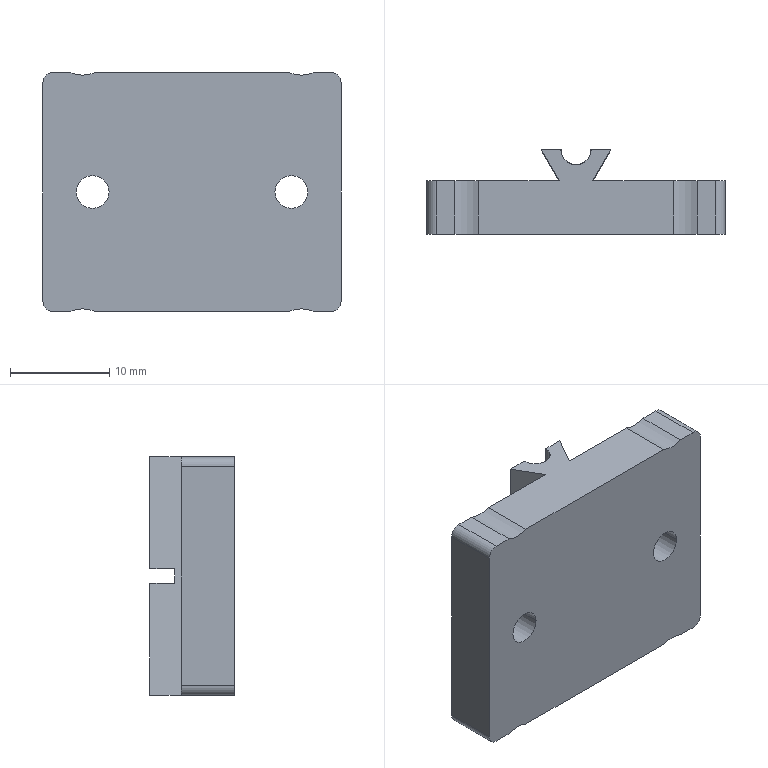Component | SolidWorks | Slider-3 | 1 solid | 39 faces | box 30 x 8.5 x 24 mm | volume 4033 mm3 | plane 20 | cylinder 14 | cone 5 | commonest cylinder face diameters 3.3 x4 2 x4 6 x4 3 x2
build123d program:
from build123d import *

# Parameters (mm, degrees)
SKETCH1_2_W                 = 24
SKETCH1_2_H                 = 30
BOSS_EXTRUDE1_DEPTH         = 10
M3_TAPPED_HOLE1_D           = 2.5
M3_TAPPED_HOLE1_CSINK_D     = 3.05
M3_TAPPED_HOLE1_CSINK_ANGLE = 100
CUT_EXTRUDE1_2_DEPTH        = 31.017
SKETCH6_W                   = 1.5
SKETCH6_H                   = 7
CUT_EXTRUDE4_DEPTH          = 4
FILLET1_R                   = 1
M4_TAPPED_HOLE3_D           = 3.3
M4_TAPPED_HOLE3_CSINK_D     = 4.05
M4_TAPPED_HOLE3_CSINK_ANGLE = 100
SKETCH1_R                   = 1.5
CUT_EXTRUDE1_DEPTH          = 24
SKETCH2_R                   = 3
CUT_EXTRUDE2_DEPTH          = 6


with BuildPart() as part:
    # Sketch1_2 → Boss-Extrude1 (new body)
    with BuildSketch(Plane(origin=(0, 0, 0), x_dir=(1, 0, 0), z_dir=(0, 1, 0))):
        Rectangle(SKETCH1_2_W, SKETCH1_2_H)
    extrude(amount=BOSS_EXTRUDE1_DEPTH)

    # M3 Tapped Hole1 (through all)
    with Locations(Plane(origin=(12, 8.5, 0), x_dir=(0, 0, 1), z_dir=(1, 0, 0))):
        with Locations((0, 0)):
            CounterSinkHole(M3_TAPPED_HOLE1_D / 2, M3_TAPPED_HOLE1_CSINK_D / 2, counter_sink_angle=M3_TAPPED_HOLE1_CSINK_ANGLE)

    # Sketch2_2 → Cut-Extrude1_2 (cut, through all)
    with BuildSketch(Plane(origin=(12, 0, 0), x_dir=(0, 0, -1), z_dir=(1, 0, 0))):
        Polygon((-15, 5.343), (-15, 10), (15, 10), (15, 5.343), (1.677, 5.343), (3.5, 8.5), (-3.5, 8.5), (-1.677, 5.343), align=None)
    extrude(amount=-CUT_EXTRUDE1_2_DEPTH, mode=Mode.SUBTRACT)

    # Sketch6 → Cut-Extrude4 (cut)
    with BuildSketch(Plane(origin=(0, 10, 0), x_dir=(1, 0, 0), z_dir=(0, 1, 0))):
        Rectangle(SKETCH6_W, SKETCH6_H)
    extrude(amount=-CUT_EXTRUDE4_DEPTH, mode=Mode.SUBTRACT)

    # Fillet1
    fillet1_edges = [part.edges().sort_by_distance(p)[0] for p in [
        (12, 2.671, 15),
        (-12, 2.671, 15),
        (-12, 2.671, -15),
        (12, 2.671, -15),
    ]]
    fillet(fillet1_edges, radius=FILLET1_R)

    # M4 Tapped Hole3 (through all)
    with Locations(Plane(origin=(0, 5.343, -10), x_dir=(0, 0, 1), z_dir=(0, 1, 0))):
        with Locations((0, 0), (20, 0)):
            CounterSinkHole(M4_TAPPED_HOLE3_D / 2, M4_TAPPED_HOLE3_CSINK_D / 2, counter_sink_angle=M4_TAPPED_HOLE3_CSINK_ANGLE)

    # Sketch1 → Cut-Extrude1 (cut)
    with BuildSketch(Plane(origin=(12, 0, 0), x_dir=(0, 0, -1), z_dir=(1, 0, 0))):
        with Locations((0, 8.5)):
            Circle(SKETCH1_R)
    extrude(amount=-CUT_EXTRUDE1_DEPTH, mode=Mode.SUBTRACT)

    # Sketch2 → Cut-Extrude2 (cut)
    with BuildSketch(Plane.XZ):
        with Locations((-14.755, 11)):
            Circle(SKETCH2_R)
        with Locations((-14.755, -11)):
            Circle(SKETCH2_R)
        with Locations((14.755, 11)):
            Circle(SKETCH2_R)
        with Locations((14.755, -11)):
            Circle(SKETCH2_R)
    extrude(amount=-CUT_EXTRUDE2_DEPTH, mode=Mode.SUBTRACT)


solid = part.part

# Placed as in the assembly
solid = solid.moved(Location((-5.981, 10.506, 234.566), (0, -90, 0)))